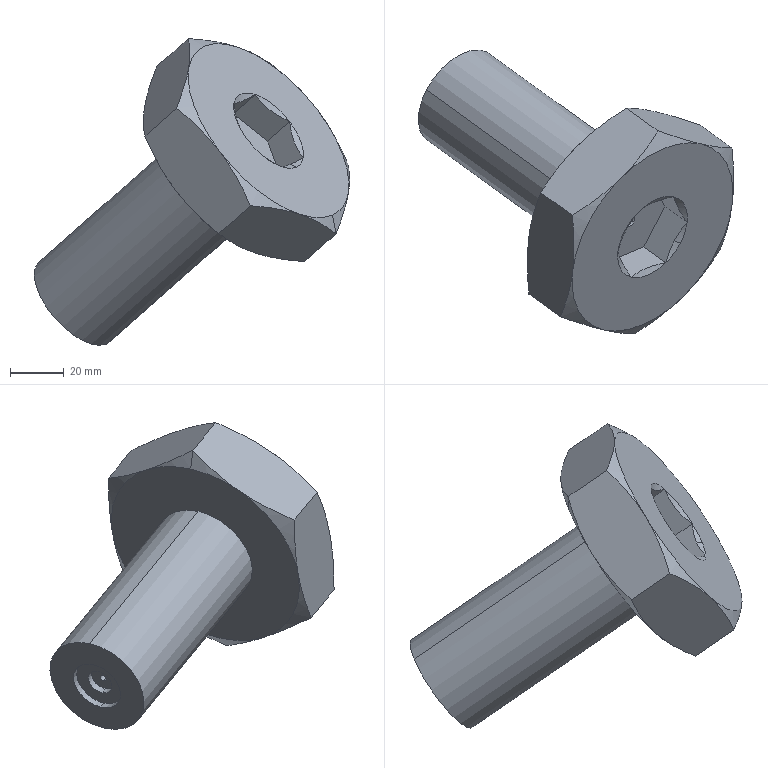Component | SolidWorks | Bolt40x60-1 | 1 solid | 49 faces | volume 233032 mm3 | cone 23 | plane 18 | cylinder 8 | commonest cylinder face diameters 20 x2 40 x2 2.4 x2 10 x2 | material Ti-3Al-8V-6Cr-4Mo-4Zr (SS)